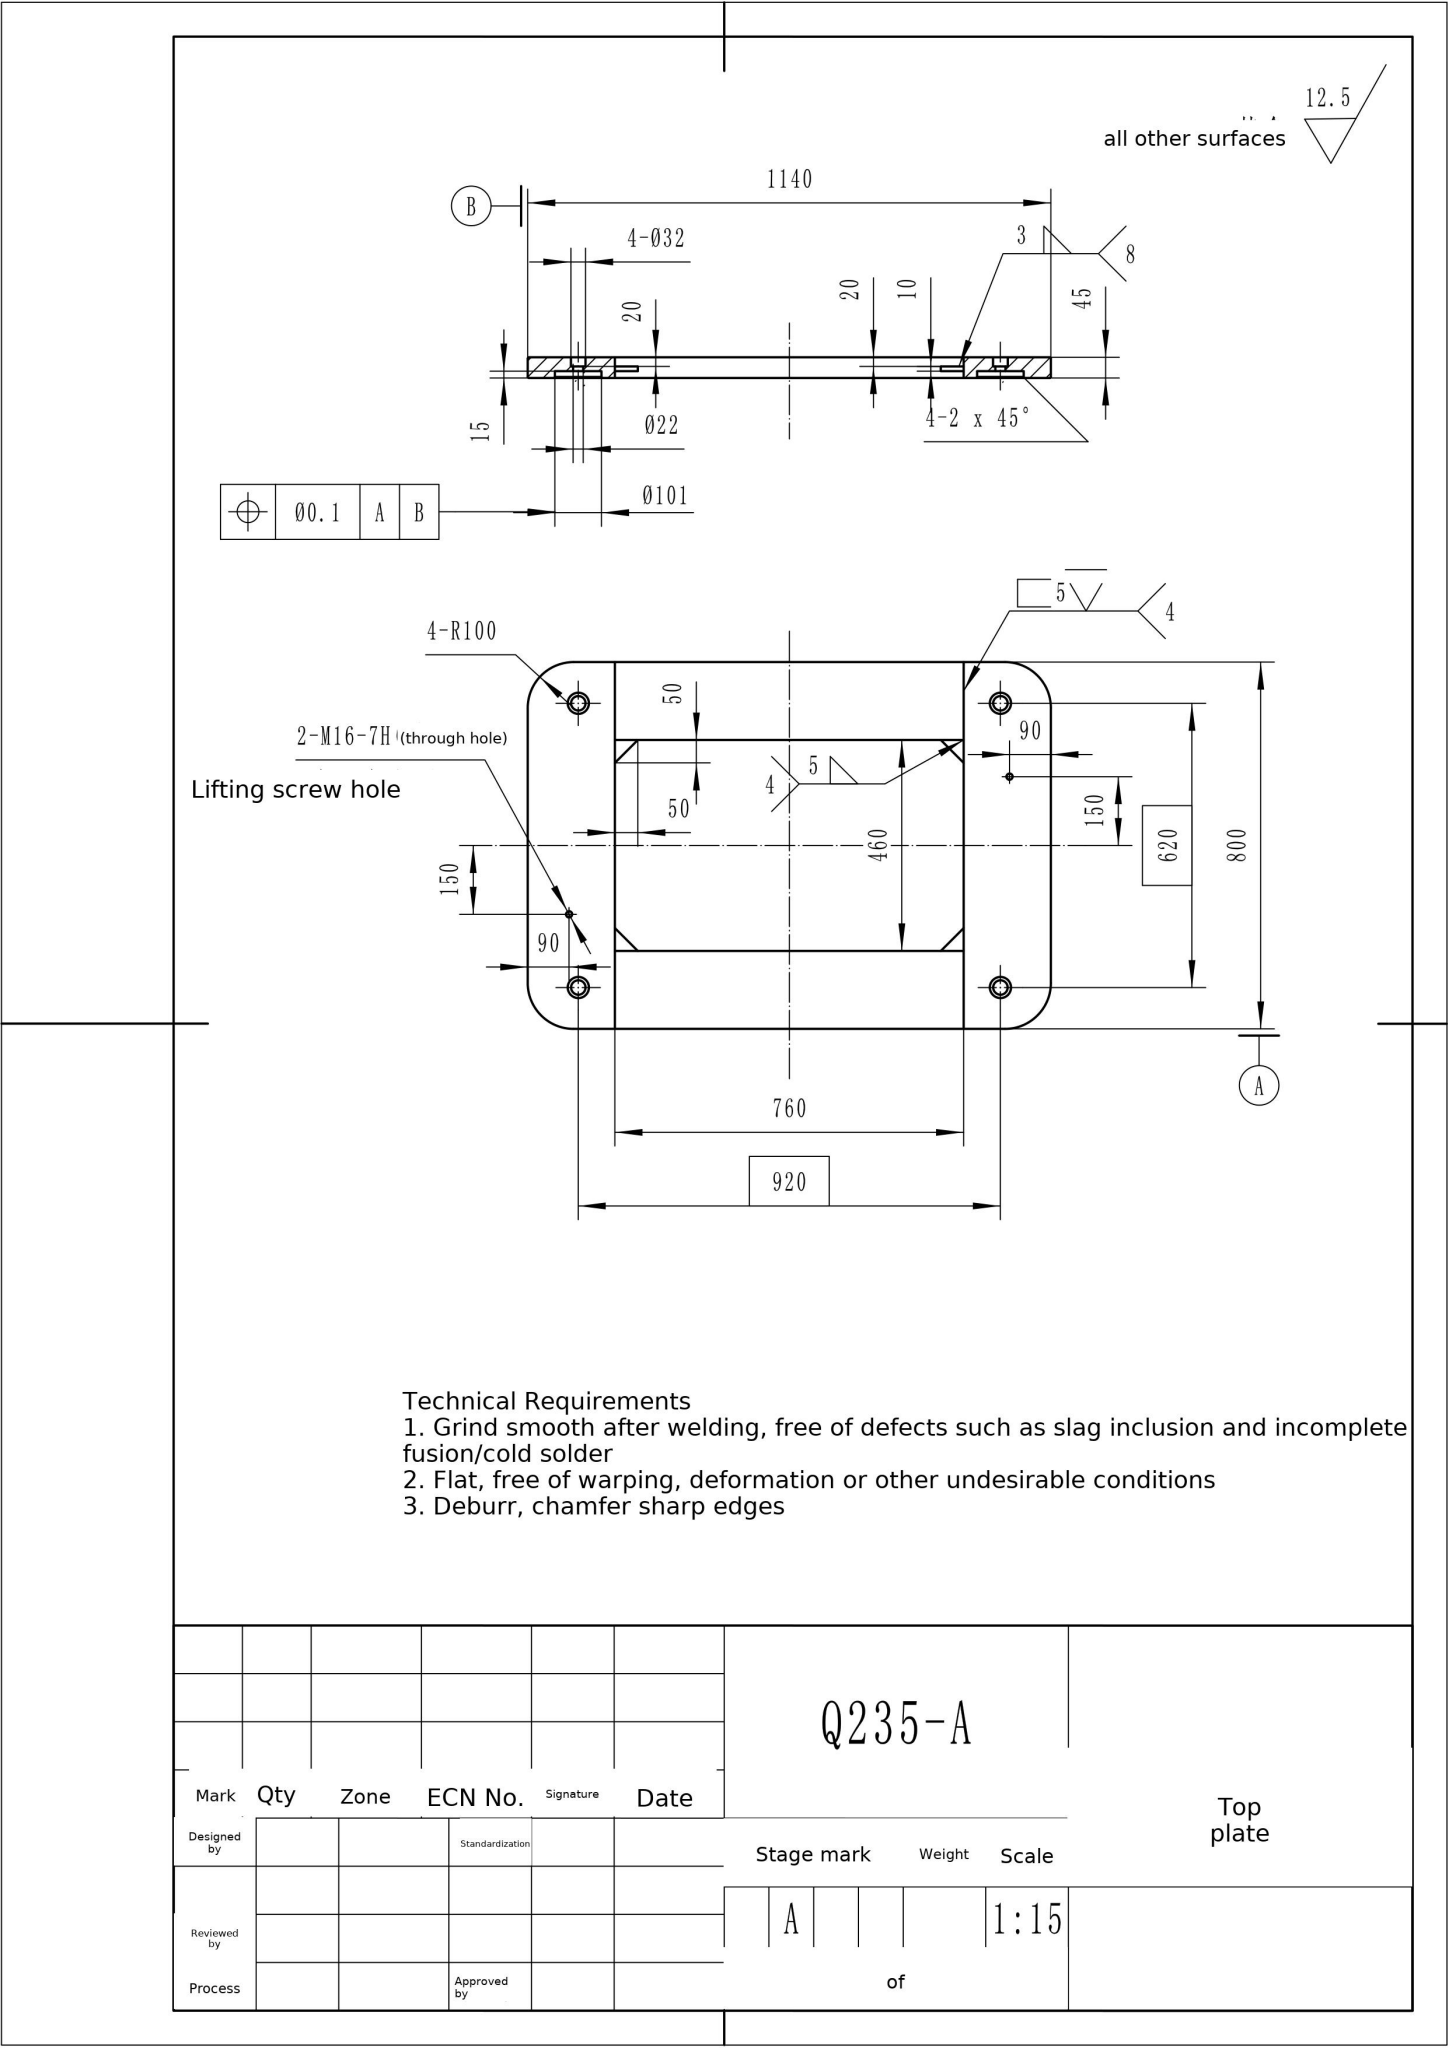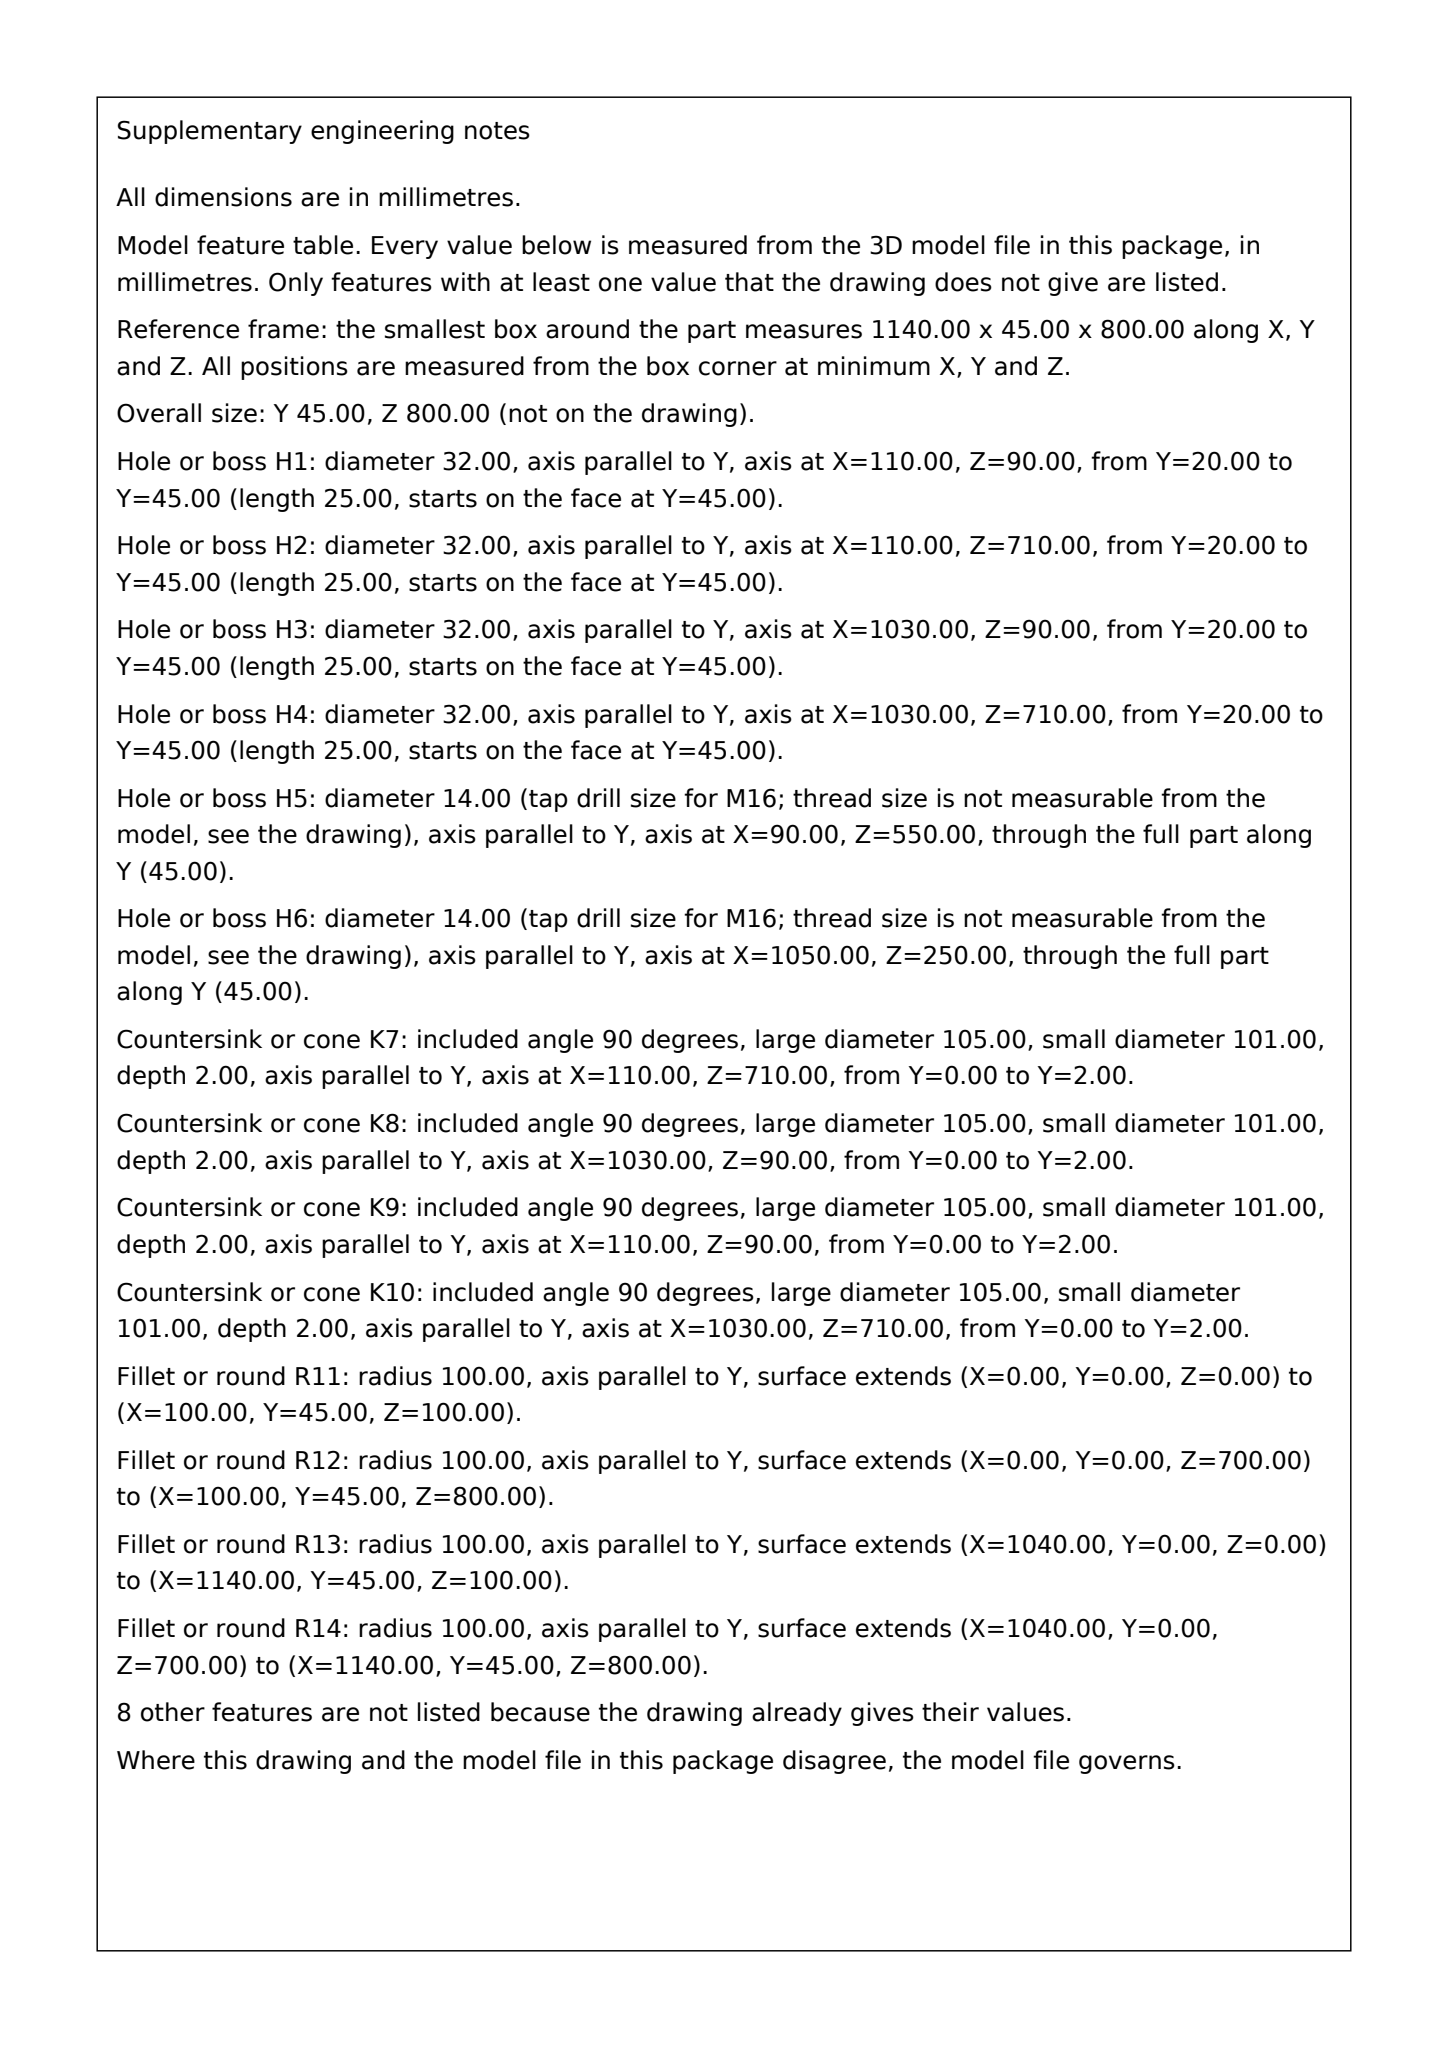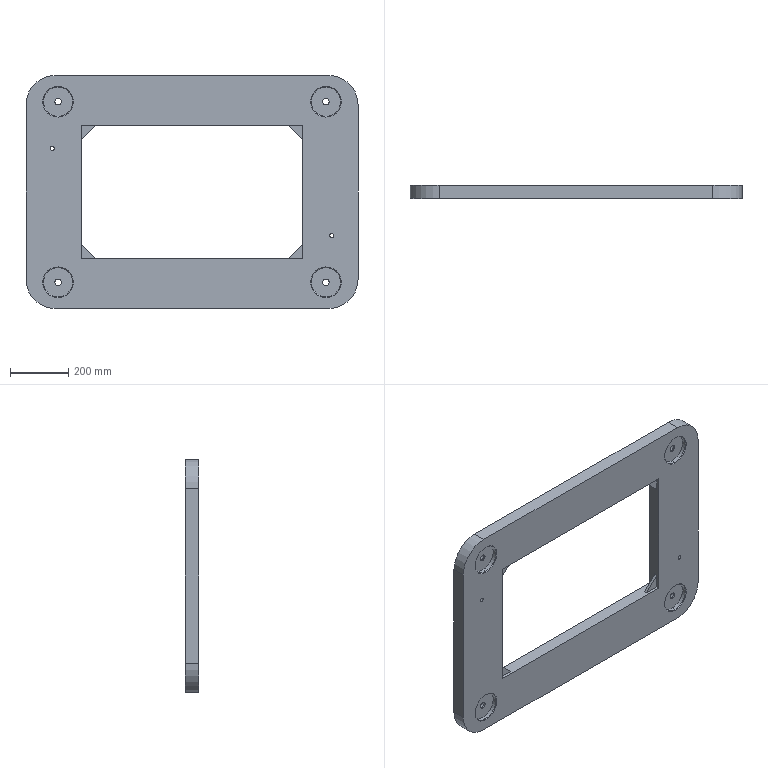Part | SolidWorks | mm | material Q235-A | 1 solid | 70 faces | box 1140 x 45 x 800 mm | volume 24386552 mm3 | cylinder 32 | plane 30 | cone 8 | commonest cylinder face diameters 101 x8 22 x8 32 x8 14 x4 200 x4
build123d program:
from build123d import *

# Parameters (mm, degrees)
SKETCH1_W                                  = 760
SKETCH1_H                                  = 460
BOSS_EXTRUDE1_DEPTH                        = 45
SKETCH3_R                                  = 16
CUT_EXTRUDE2_DEPTH                         = 25
SKETCH4_R                                  = 11
CUT_EXTRUDE3_DEPTH                         = 698.8
CUT_EXTRUDE4_START                         = -45
SKETCH5_R                                  = 50.5
CUT_EXTRUDE4_DEPTH                         = 15
BOSS_EXTRUDE2_START                        = -35
BOSS_EXTRUDE2_DEPTH                        = 10
MIRROR1_AT_THE_SECOND_PLANE_COPY_1_SKETC_R = 16
MIRROR1_AT_THE_SECOND_PLANE_COPY_1_DEPTH   = 25
MIRROR1_AT_THE_SECOND_PLANE_COPY_2_SKETC_R = 11
MIRROR1_AT_THE_SECOND_PLANE_COPY_2_DEPTH   = 698.8
MIRROR1_START                              = -45
MIRROR1_AT_THE_SECOND_PLANE_COPY_3_SKETC_R = 50.5
MIRROR1_AT_THE_SECOND_PLANE_COPY_3_DEPTH   = 15
MIRROR1_START_2                            = -35
MIRROR1_AT_THE_SECOND_PLANE_COPY_4_DEPTH   = 10
M16_TAPPED_HOLE1_D                         = 14
CHAMFER1_SIZE                              = 2


with BuildPart() as part:
    # Sketch1 → Boss-Extrude1 (new body)
    with BuildSketch(Plane(origin=(0, 0, 0), x_dir=(1, 0, 0), z_dir=(0, 1, 0))):
        with BuildLine():
            Line((-470, -400), (470, -400))
            ThreePointArc((470, -400), (540.711, -370.711), (570, -300))
            Line((570, -300), (570, 300))
            ThreePointArc((570, 300), (540.711, 370.711), (470, 400))
            Line((470, 400), (-470, 400))
            ThreePointArc((-470, 400), (-540.711, 370.711), (-570, 300))
            Line((-570, 300), (-570, -300))
            ThreePointArc((-570, -300), (-540.711, -370.711), (-470, -400))
        make_face()
        Rectangle(SKETCH1_W, SKETCH1_H, mode=Mode.SUBTRACT)
    extrude(amount=-BOSS_EXTRUDE1_DEPTH)

    # Sketch3 → Cut-Extrude2 (cut)
    with BuildSketch(Plane(origin=(0, 0, 0), x_dir=(1, 0, 0), z_dir=(0, 1, 0))):
        with Locations(Location((-460, 310, 0), (0, 0, 270))):
            Circle(SKETCH3_R)
    cut_extrude2 = extrude(amount=-CUT_EXTRUDE2_DEPTH, mode=Mode.SUBTRACT)

    # Sketch4 → Cut-Extrude3 (cut, through all)
    with BuildSketch(Plane(origin=(0, 0, 0), x_dir=(1, 0, 0), z_dir=(0, 1, 0))):
        with Locations(Location((-460, 310, 0), (0, 0, 270))):
            Circle(SKETCH4_R)
    cut_extrude3 = extrude(amount=-CUT_EXTRUDE3_DEPTH, mode=Mode.SUBTRACT)

    # Sketch5 → Cut-Extrude4 (cut)
    with BuildSketch(Plane(origin=(0, 0, 0), x_dir=(1, 0, 0), z_dir=(0, 1, 0)).offset(CUT_EXTRUDE4_START)):
        with Locations(Location((-460, 310, 0), (0, 0, 270))):
            Circle(SKETCH5_R)
    cut_extrude4 = extrude(amount=CUT_EXTRUDE4_DEPTH, mode=Mode.SUBTRACT)

    # Sketch6 → Boss-Extrude2 (add)
    with BuildSketch(Plane(origin=(0, 0, 0), x_dir=(1, 0, 0), z_dir=(0, 1, 0)).offset(BOSS_EXTRUDE2_START)):
        Polygon((-330, 230), (-380, 180), (-380, 230), align=None)
    boss_extrude2 = extrude(amount=BOSS_EXTRUDE2_DEPTH)

    # Mirror1: Cut-Extrude2, Cut-Extrude3, Cut-Extrude4, Boss-Extrude2 across plane
    add(cut_extrude2.mirror(Plane(origin=(0, 0, 0), x_dir=(0, 0, 1), z_dir=(1, 0, 0))), mode=Mode.SUBTRACT)
    add(cut_extrude3.mirror(Plane(origin=(0, 0, 0), x_dir=(0, 0, 1), z_dir=(1, 0, 0))), mode=Mode.SUBTRACT)
    add(cut_extrude4.mirror(Plane(origin=(0, 0, 0), x_dir=(0, 0, 1), z_dir=(1, 0, 0))), mode=Mode.SUBTRACT)
    add(boss_extrude2.mirror(Plane(origin=(0, 0, 0), x_dir=(0, 0, 1), z_dir=(1, 0, 0))))

    # Mirror1 at the second plane: Cut-Extrude2, Cut-Extrude3, Cut-Extrude4, Boss-Extrude2 across plane
    add(cut_extrude2.mirror(Plane.XY), mode=Mode.SUBTRACT)
    add(cut_extrude3.mirror(Plane.XY), mode=Mode.SUBTRACT)
    add(cut_extrude4.mirror(Plane.XY), mode=Mode.SUBTRACT)
    add(boss_extrude2.mirror(Plane.XY))

    # Mirror1 at the second plane copy 1 sketc → Mirror1 at the second plane copy 1 (cut)
    with BuildSketch(Plane(origin=(0, 0, 0), x_dir=(-1, 0, 0), z_dir=(0, 1, 0))):
        with Locations(Location((-460, 310, 0), (0, 0, 270))):
            Circle(MIRROR1_AT_THE_SECOND_PLANE_COPY_1_SKETC_R)
    extrude(amount=-MIRROR1_AT_THE_SECOND_PLANE_COPY_1_DEPTH, mode=Mode.SUBTRACT)

    # Mirror1 at the second plane copy 2 sketc → Mirror1 at the second plane copy 2 (cut, through all)
    with BuildSketch(Plane(origin=(0, 0, 0), x_dir=(-1, 0, 0), z_dir=(0, 1, 0))):
        with Locations(Location((-460, 310, 0), (0, 0, 270))):
            Circle(MIRROR1_AT_THE_SECOND_PLANE_COPY_2_SKETC_R)
    extrude(amount=-MIRROR1_AT_THE_SECOND_PLANE_COPY_2_DEPTH, mode=Mode.SUBTRACT)

    # Mirror1 at the second plane copy 3 sketc → Mirror1 at the second plane copy 3 (cut)
    with BuildSketch(Plane(origin=(0, 0, 0), x_dir=(-1, 0, 0), z_dir=(0, 1, 0)).offset(MIRROR1_START)):
        with Locations(Location((-460, 310, 0), (0, 0, 270))):
            Circle(MIRROR1_AT_THE_SECOND_PLANE_COPY_3_SKETC_R)
    extrude(amount=MIRROR1_AT_THE_SECOND_PLANE_COPY_3_DEPTH, mode=Mode.SUBTRACT)

    # Mirror1 at the second plane copy 4 sketc → Mirror1 at the second plane copy 4 (add)
    with BuildSketch(Plane(origin=(0, 0, 0), x_dir=(-1, 0, 0), z_dir=(0, 1, 0)).offset(MIRROR1_START_2)):
        Polygon((-330, 230), (-380, 180), (-380, 230), align=None)
    extrude(amount=MIRROR1_AT_THE_SECOND_PLANE_COPY_4_DEPTH)

    # M16 Tapped Hole1 (through all)
    with Locations(Plane(origin=(-480, 0, 150), x_dir=(0, 0, 1), z_dir=(0, 1, 0))):
        with Locations((0, 0), (-300, 960)):
            Hole(M16_TAPPED_HOLE1_D / 2)

    # Chamfer1
    chamfer1_edges = [part.edges().sort_by_distance(p)[0] for p in [
        (460, -45, -360.5),
        (460, -45, 360.5),
        (-460, -45, -360.5),
        (-460, -45, 360.5),
    ]]
    chamfer(chamfer1_edges, length=CHAMFER1_SIZE)


solid = part.part